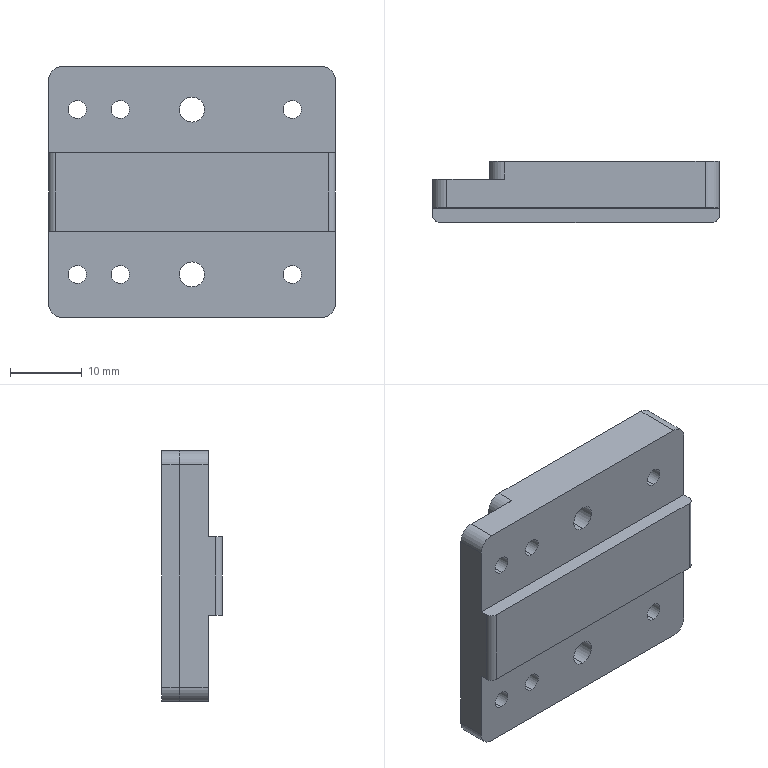CAM job | Mastercam | mm | 15 operations | part box 40 x 8.5 x 35
1. Facing | 20 - 63 平铣刀
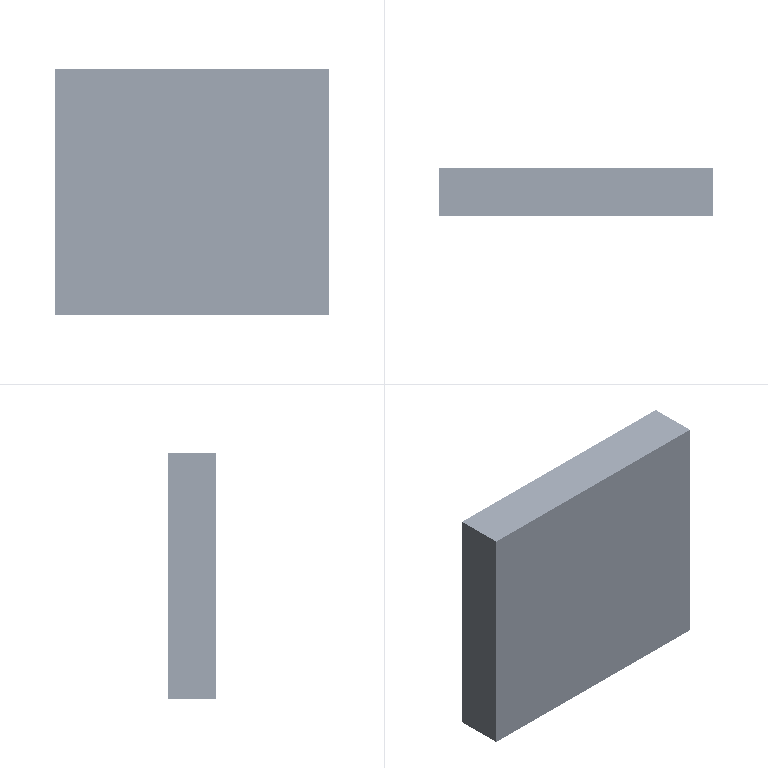2. Contour (Ramp) | 12 - 12 平铣刀
3. Contour (Ramp) | 12 - 12 平铣刀
4. Surface Finish Flowline | 9 - 8 圆鼻铣刀
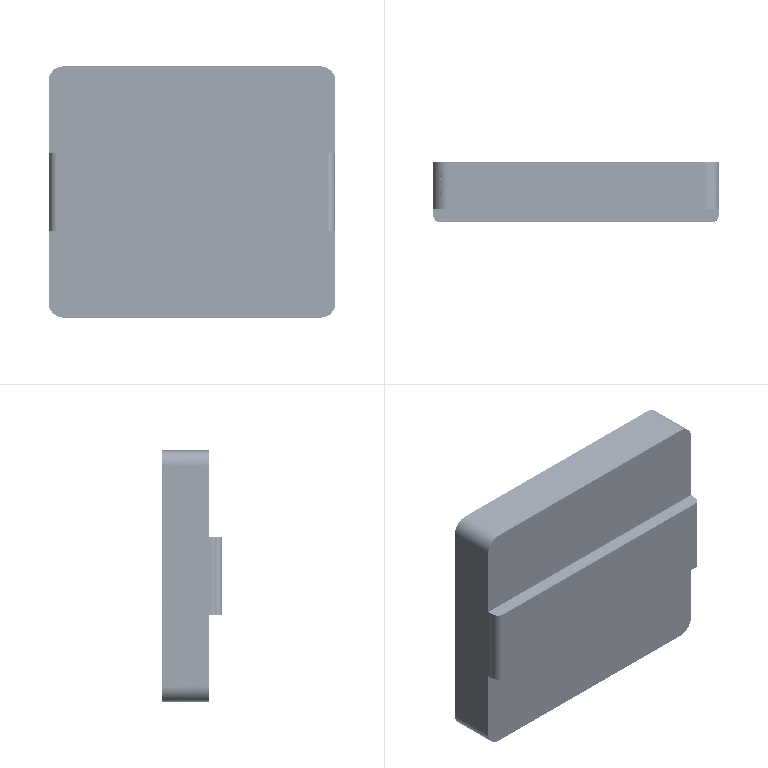5. Contour (2D) | 10 - 10 平铣刀
6. Contour (2D) | 10 - 10 平铣刀
7. Drill/Counterbore | 7 - 4 倒角刀
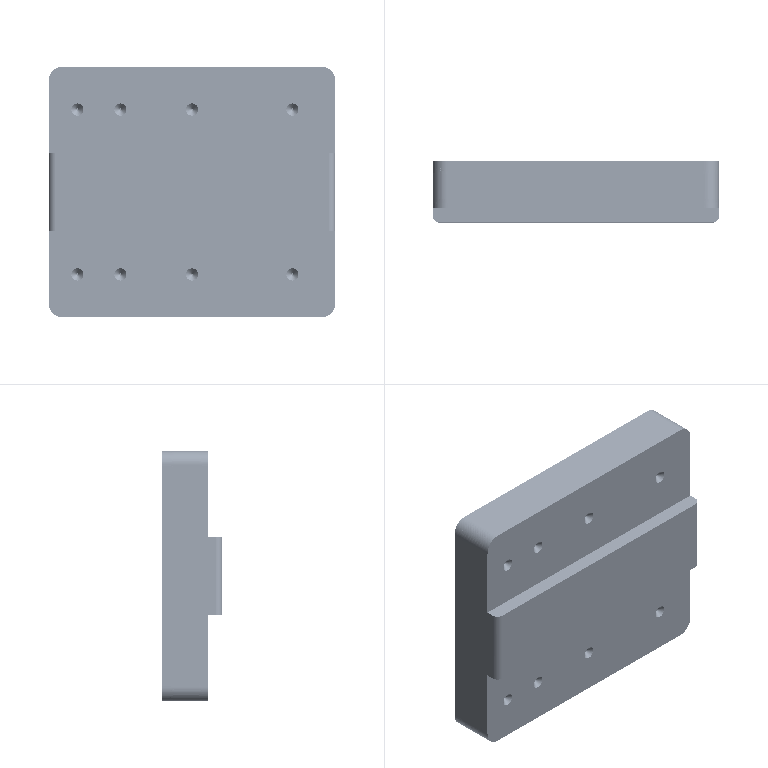8. Deburr 5-axis | 3 - 3 球刀/圆鼻铣刀
9. Facing | 20 - 63 平铣刀
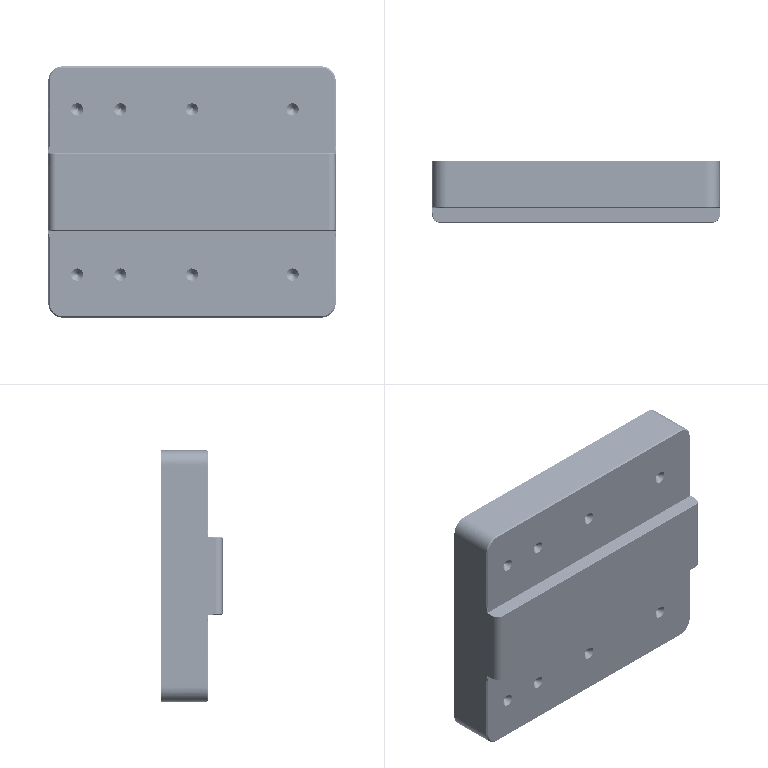10. Contour (Ramp) | 12 - 12 平铣刀
11. Contour (2D) | 10 - 10 平铣刀
12. Contour (2D) | 10 - 10 平铣刀
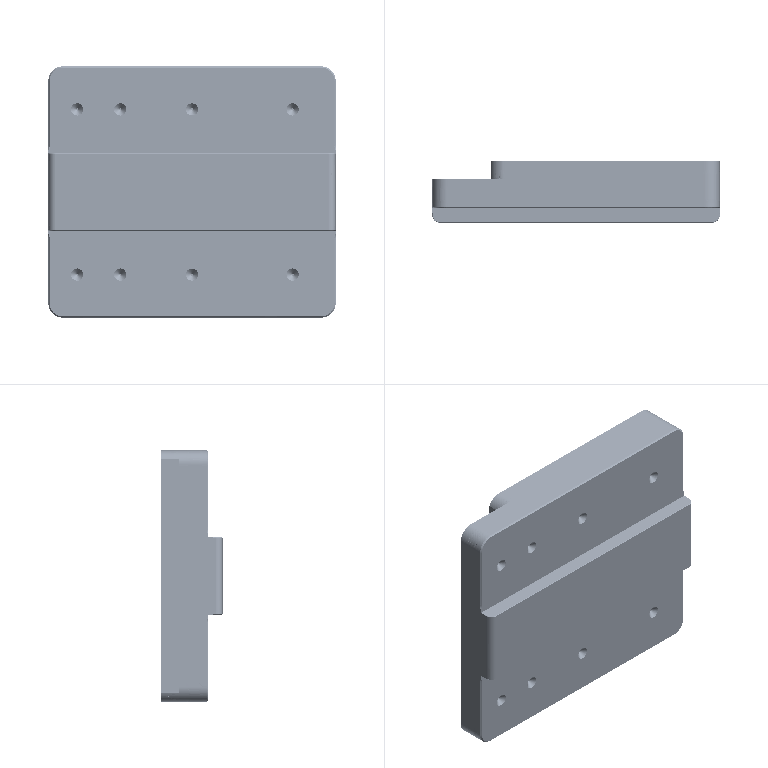13. Contour (Ramp) | 4 - 4 平铣刀
14. Contour (2D) | 4 - 4 平铣刀
15. Deburr 5-axis | 3 - 3 球刀/圆鼻铣刀